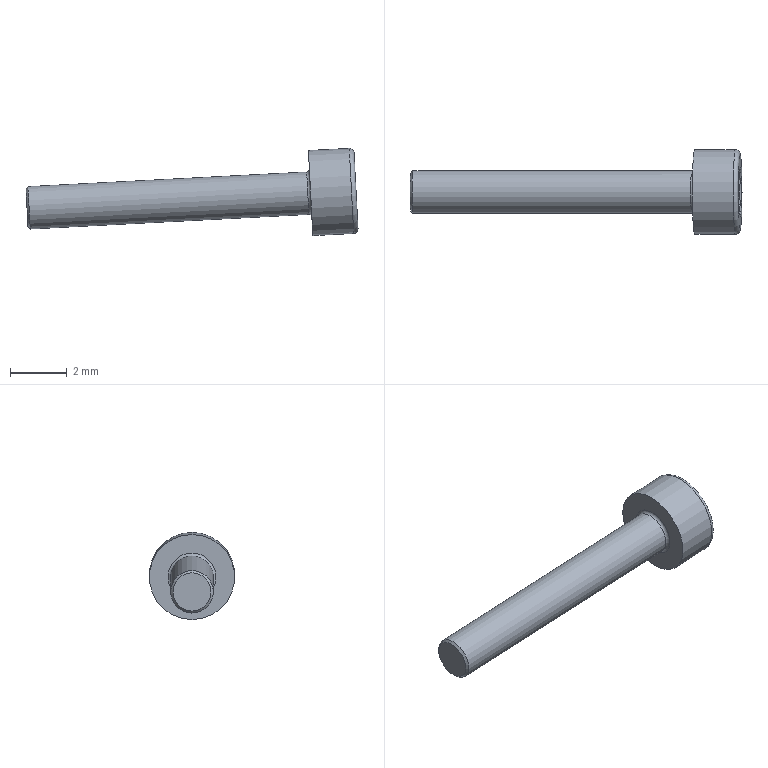Component | NX | GB-T70_1-2000_M1_6X10_2 | 1 solid | 27 faces | volume 27 mm3 | plane 15 | cone 8 | cylinder 2 | torus 2 | commonest cylinder face diameters 1.496 x1 3 x1